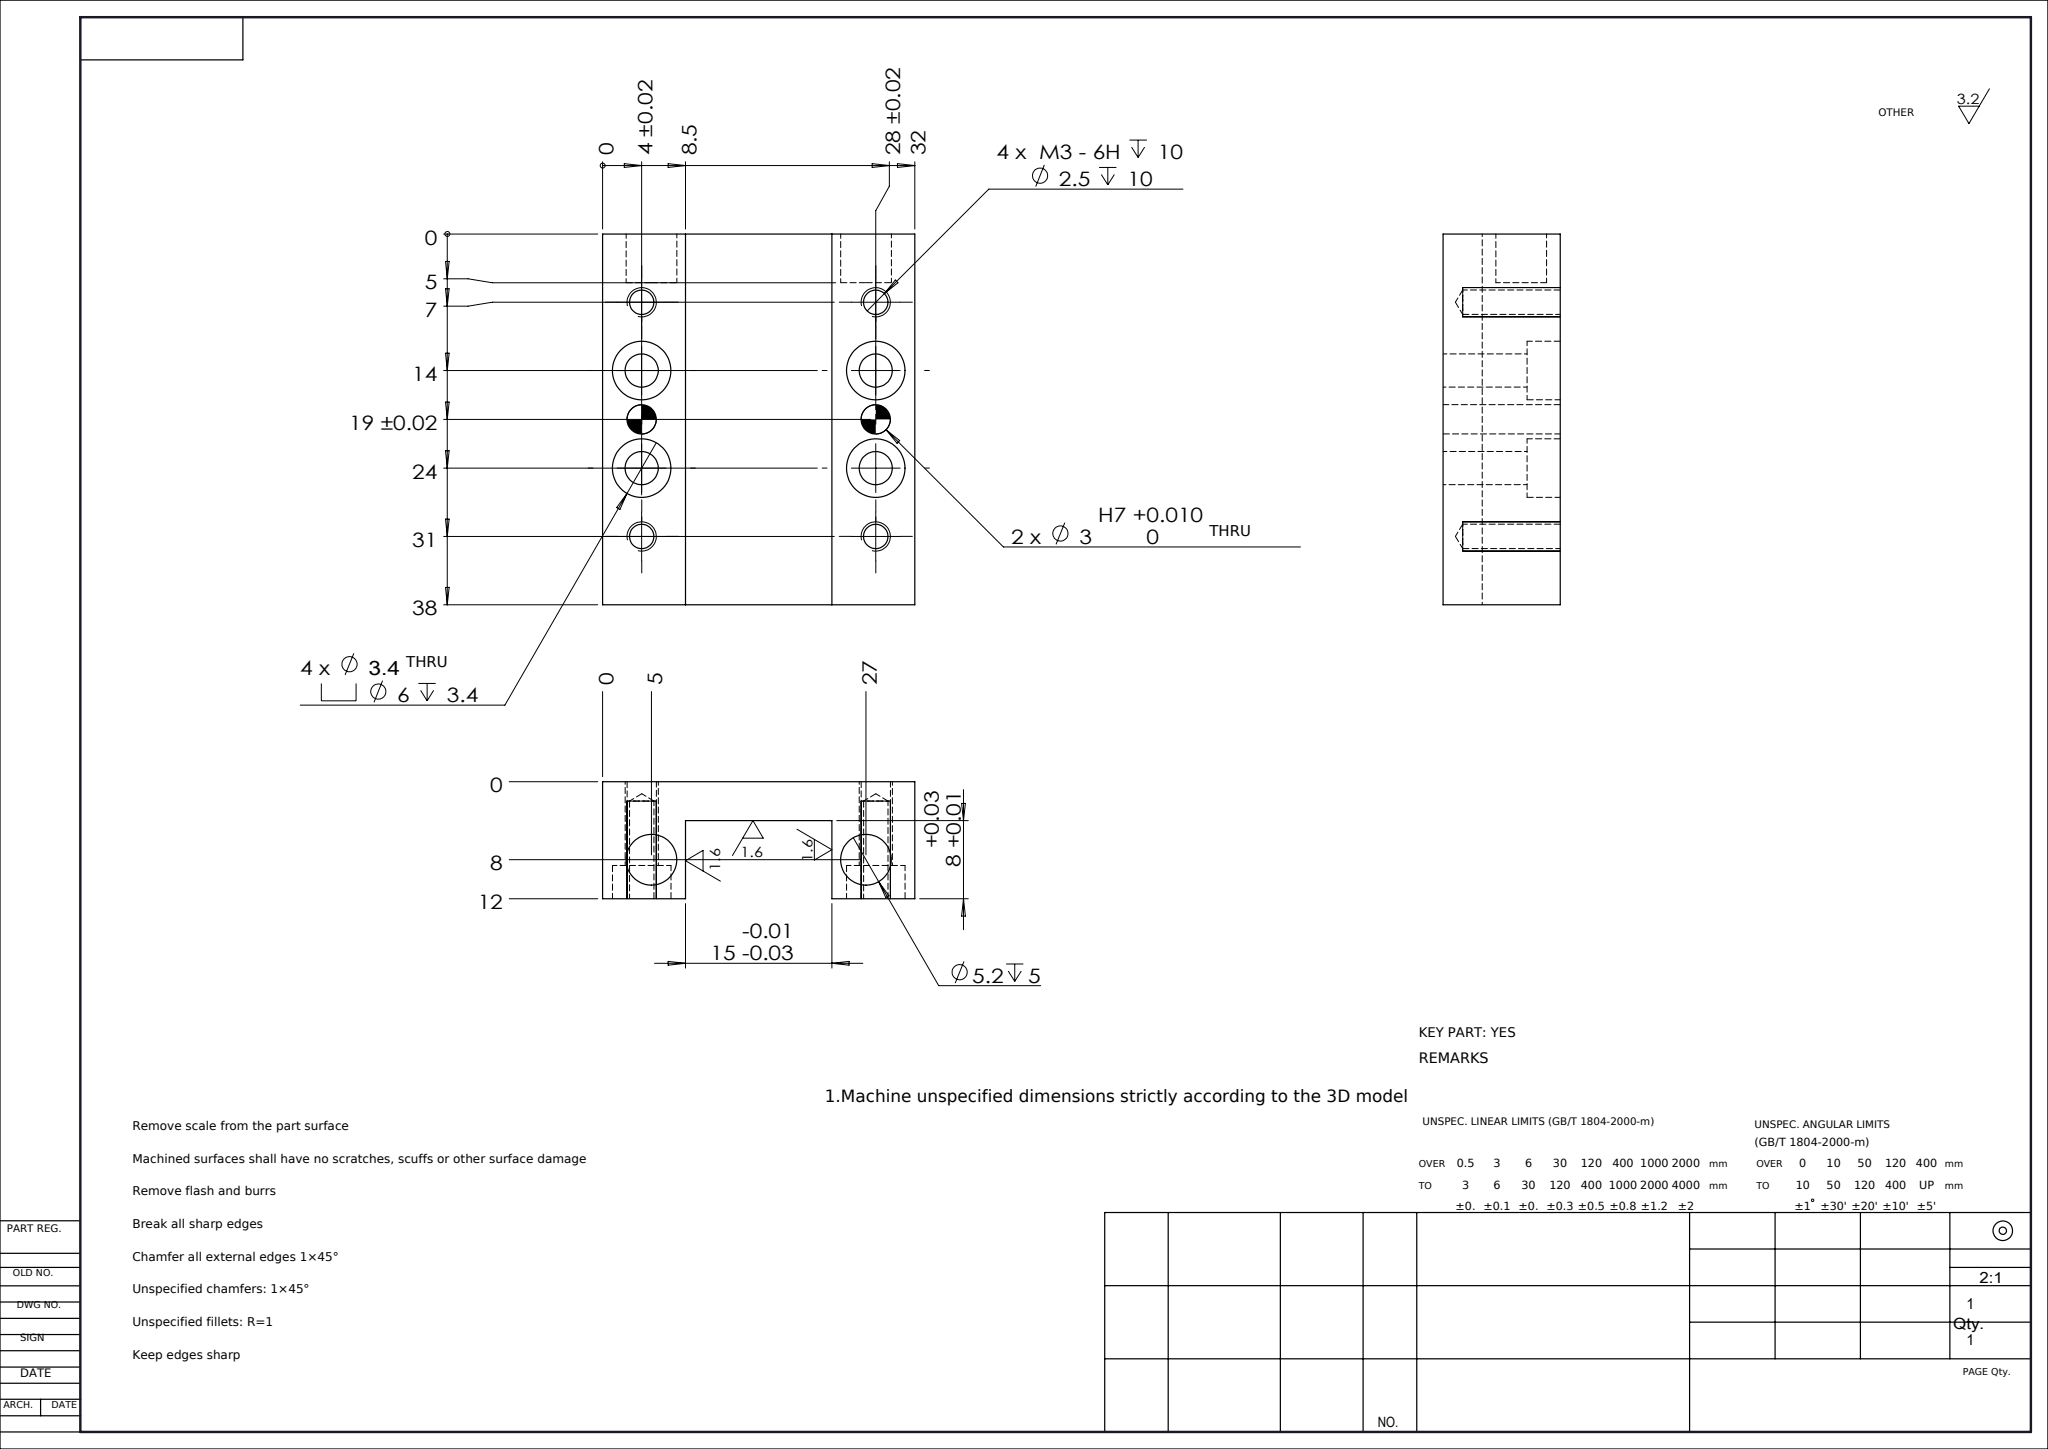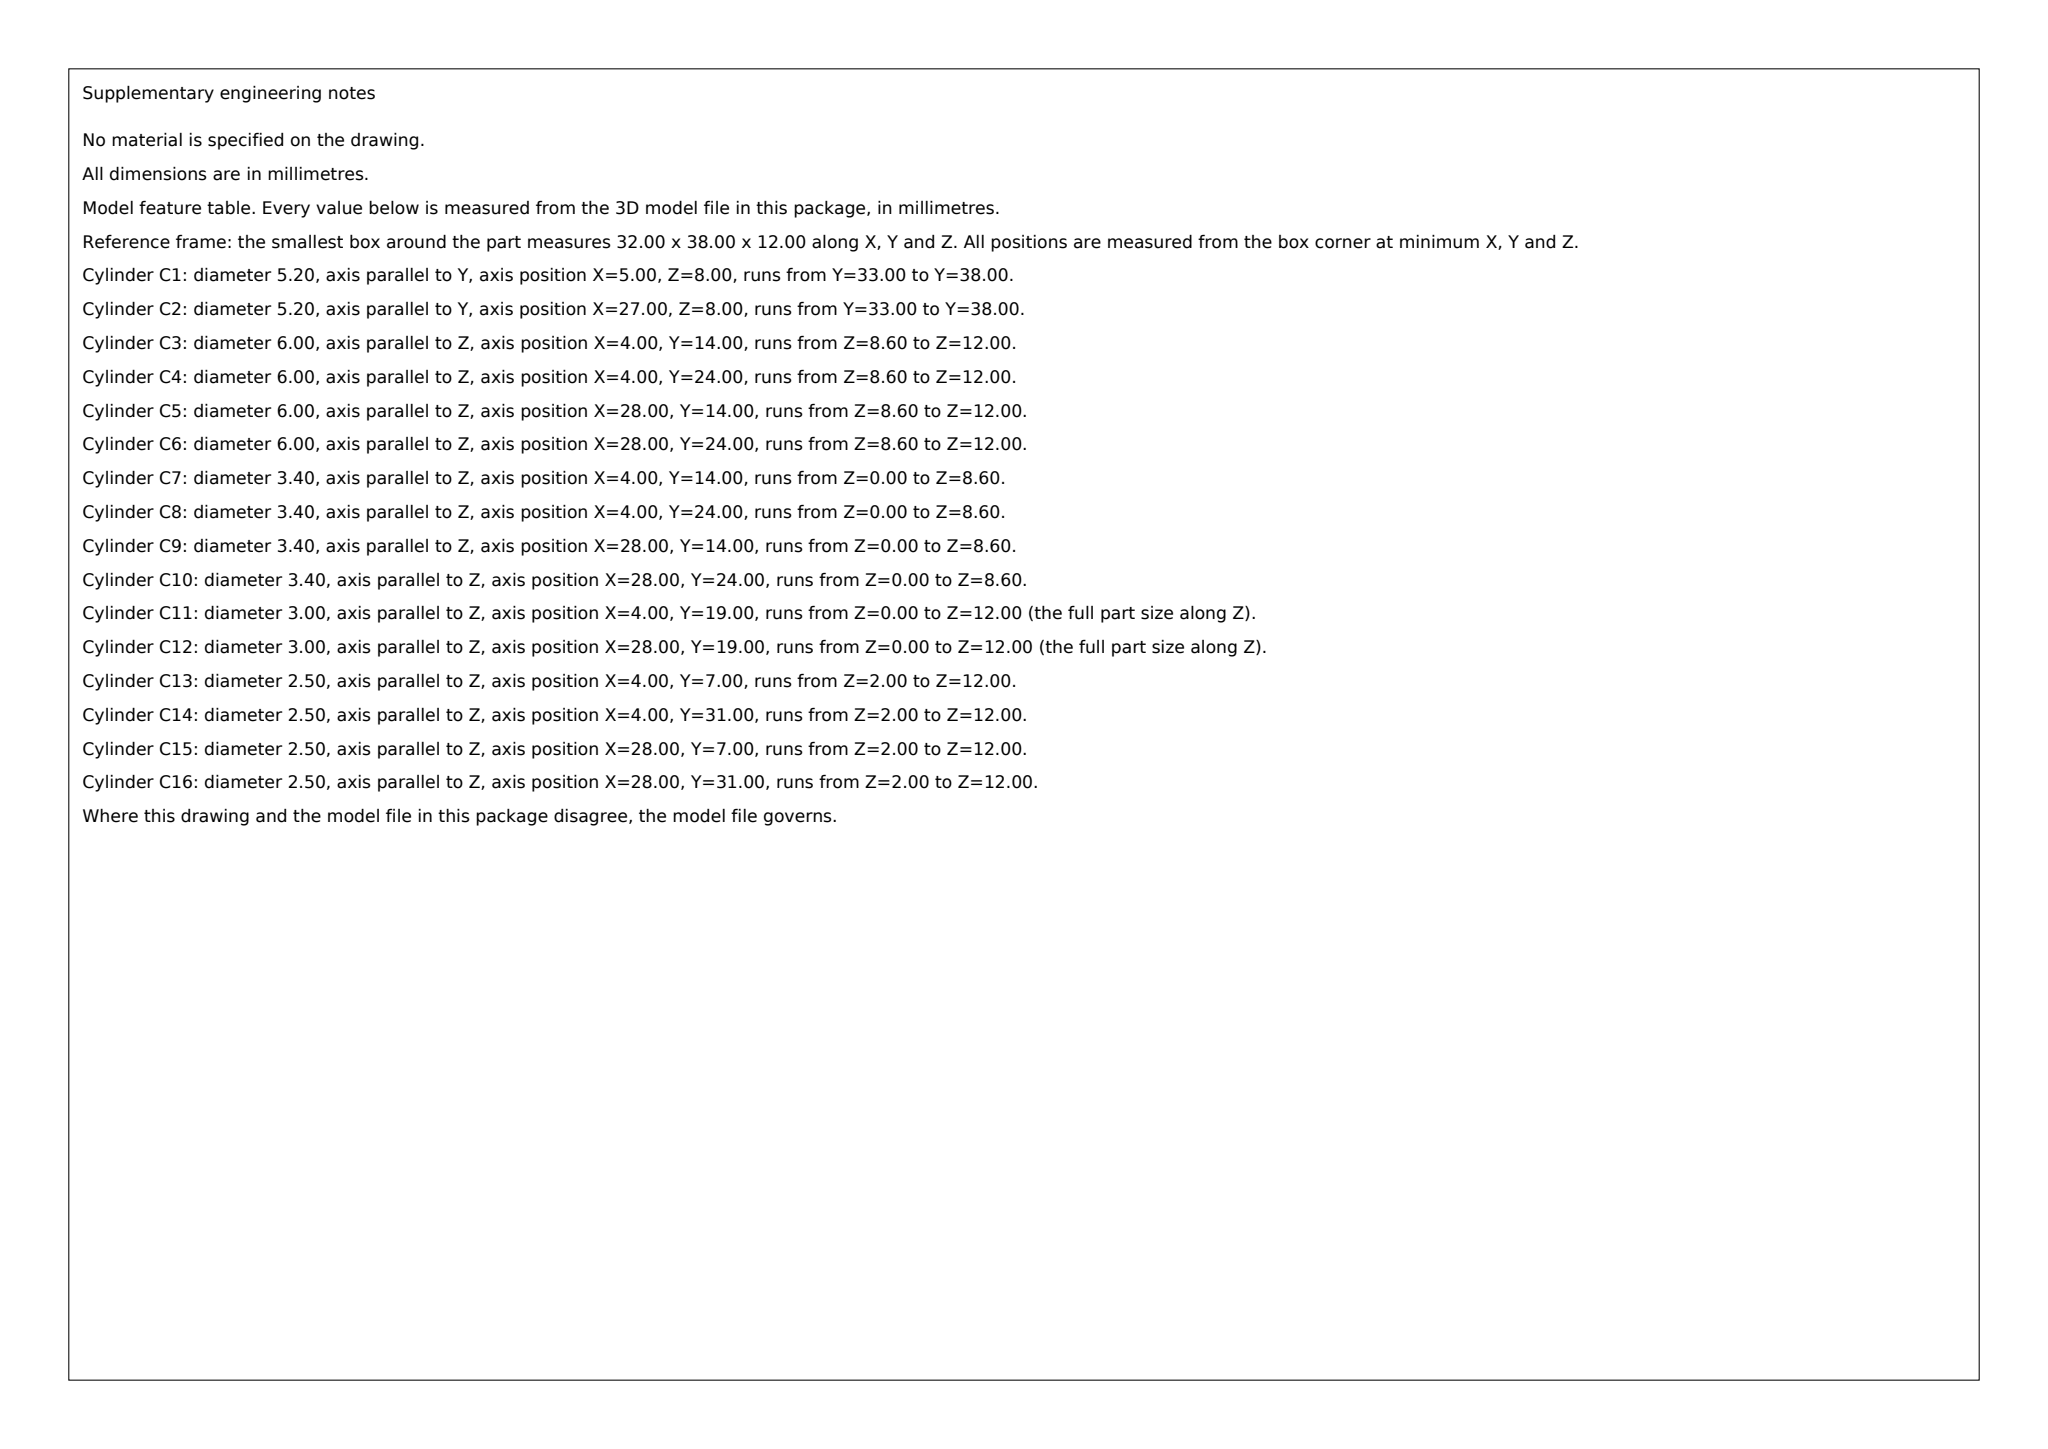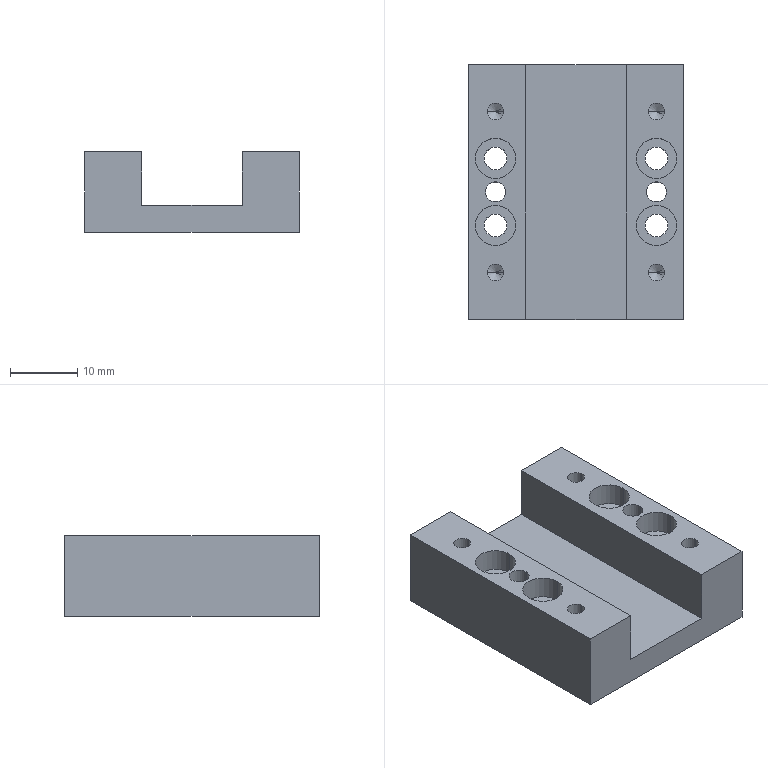Part | SolidWorks | mm | 1 solid | 56 faces | box 32 x 38 x 12 mm | volume 8752 mm3 | cylinder 32 | plane 16 | cone 8 | commonest cylinder face diameters 2.5 x8 6 x8 3.4 x8 3 x4 5.2 x4
build123d program:
from build123d import *

# Parameters (mm, degrees)
SKETCH1_W                                         = 32
SKETCH1_H                                         = 38
BOSS_EXTRUDE1_DEPTH                               = 12
SKETCH3_W                                         = 15
SKETCH3_H                                         = 8
CUT_EXTRUDE2_DEPTH                                = 38
SKETCH5_R                                         = 2.6
CUT_EXTRUDE3_DEPTH                                = 5
HOLE_SIZE_ACCORDING_TO_HEXAGON_SOCKET_D           = 3.4
HOLE_SIZE_ACCORDING_TO_HEXAGON_SOCKET_CBORE_D     = 6
HOLE_SIZE_ACCORDING_TO_HEXAGON_SOCKET_CBORE_DEPTH = 3.4
SIZE_MM_DOWEL_PIN_HOLE_1_D                        = 3
M3_TAPPED_HOLE1_D                                 = 2.5
M3_TAPPED_HOLE1_DEPTH                             = 10
M3_TAPPED_HOLE1_TIP                               = 0.7511


with BuildPart() as part:
    # Sketch1 → Boss-Extrude1 (new body)
    with BuildSketch(Plane.XY):
        Rectangle(SKETCH1_W, SKETCH1_H)
    extrude(amount=BOSS_EXTRUDE1_DEPTH)

    # Sketch3 → Cut-Extrude2 (cut)
    with BuildSketch(Plane.XZ.offset(19)):
        with Locations((0, 8)):
            Rectangle(SKETCH3_W, SKETCH3_H)
    extrude(amount=-CUT_EXTRUDE2_DEPTH, mode=Mode.SUBTRACT)

    # Sketch5 → Cut-Extrude3 (cut)
    with BuildSketch(Plane(origin=(0, 19, 0), x_dir=(1, 0, 0), z_dir=(0, 1, 0))):
        with Locations(Location((11, -8, 0), (0, 0, 270))):
            Circle(SKETCH5_R)
        with Locations(Location((-11, -8, 0), (0, 0, 270))):
            Circle(SKETCH5_R)
    extrude(amount=-CUT_EXTRUDE3_DEPTH, mode=Mode.SUBTRACT)

    # Hole Size _ according to_ Hexagon Socket (through all)
    with Locations(Plane.XY.offset(12)):
        with Locations((12, 5), (-12, 5), (-12, -5), (12, -5)):
            CounterBoreHole(HOLE_SIZE_ACCORDING_TO_HEXAGON_SOCKET_D / 2, HOLE_SIZE_ACCORDING_TO_HEXAGON_SOCKET_CBORE_D / 2, HOLE_SIZE_ACCORDING_TO_HEXAGON_SOCKET_CBORE_DEPTH)

    # Size mm Dowel Pin Hole 1 (through all)
    with Locations(Plane.XY.offset(12)):
        with Locations((12, 0), (-12, 0)):
            Hole(SIZE_MM_DOWEL_PIN_HOLE_1_D / 2)

    # M3 Tapped Hole1
    with Locations(Plane.XY.offset(12)):
        with Locations((12, 12), (-12, 12), (-12, -12), (12, -12)):
            Hole(M3_TAPPED_HOLE1_D / 2, depth=M3_TAPPED_HOLE1_DEPTH)
            with Locations((0, 0, -(M3_TAPPED_HOLE1_DEPTH + M3_TAPPED_HOLE1_TIP / 2))):  # 118° drill point
                Cone(0, M3_TAPPED_HOLE1_D / 2, M3_TAPPED_HOLE1_TIP, mode=Mode.SUBTRACT)


solid = part.part